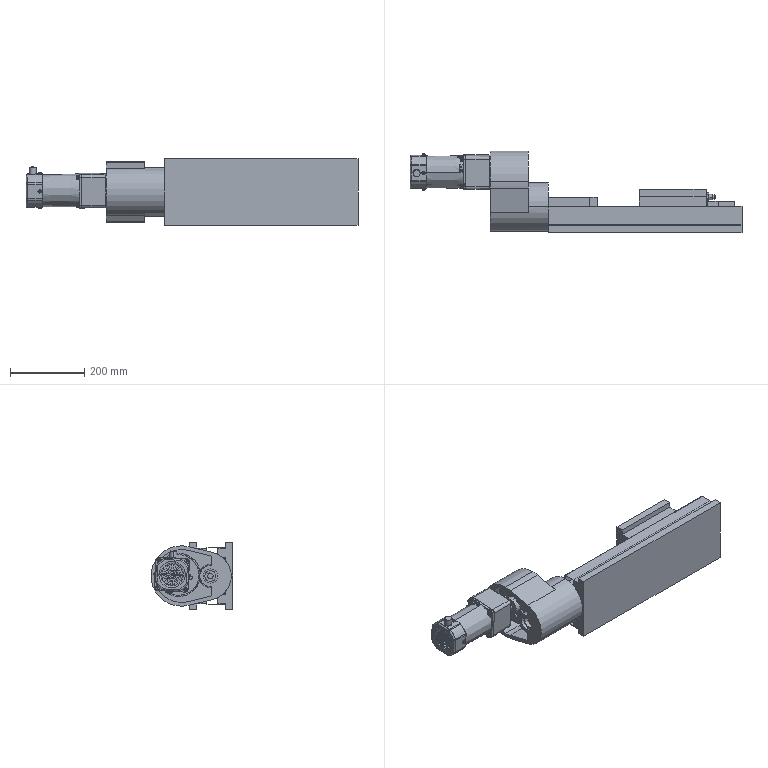Assembly | SolidWorks | mm | 44 component files | 275 solids | 3085 faces | box 892.1 x 219.71 x 180 mm | volume 7665810 mm3 | cylinder 1026 | sphere 846 | plane 710 | spline 244 | cone 147 | torus 112 | commonest cylinder face diameters 115.5 x76 108.75 x75 2 x53 20 x52 15 x47 39 x38 50.25 x36 57 x36
Bill of materials:
BallScrew | 1 |  | Long, slender cylindrical shaft. Both ends step down to smaller diameters, and there is a band of evenly spaced circumferential grooves partway along its length.
BearingHousing | 1 |  | Appears to be two separate prismatic bodies. One is a thin rectangular block with a round through-hole and a recessed or open lower region. The other is a solid rectangular box next to it.
ConnectingFlange | 2 |  | Long, straight, thin-walled profile with a Z/S-shaped cross-section. Two parallel flanges are joined by a web, with rounded bends at the corners.
ConnectingSeat | 1 |  | Rectangular block with a large cylindrical through-bore. Seen from the end, it has a stepped T-like profile: a wider flange section on one side and a narrower body around the bore.
CopperGasket | 1 |  | Thin flat rectangular plate with four small round through-holes in a rectangular pattern, set in from the edges.
CountersunkScrewM5X20 | 6 |  | Stepped cylindrical pin. A larger-diameter head transitions to a smaller shank with a chamfered end, and there is a polygonal socket recess in the head end face.
CountersunkScrewM8x4 | 4 |  | Stepped cylindrical pin with a short, larger-diameter head and a longer, smaller-diameter shank that has a chamfered tip.
CouplingSleeve | 1 |  | Cylindrical tube or sleeve with a coaxial bore. There is a small rectangular notch or keyway-like cut in the bore wall along its length.
DeepGrooveBallBearing16002 | 5 |  | Ring-shaped assembly-like body with an outer ring, a wide inner ring with a central bore, and a single circular row of balls between them.
DeepGrooveBallBearing6204 | 1 |  | Thin-section ring body with narrow outer and inner rings, a single circular row of balls between them, and a large central opening.
EndCap | 1 |  | Bracket-like body: a flat rectangular plate with four corner holes and a rectangular slot, with a hollow rectangular frame extending from one face. Curved surfaces are visible inside the frame.
Gearbox | 1 |  | Stepped solid with a teardrop/obround (cam-like) profile: a large rounded lobe joined to a smaller rounded end by tangent flats. It has a small through-hole near the smaller end and a thickness step between regions.
GearboxLargeGear | 1 |  | Straight-toothed spur gear with many teeth, a central round bore, six round holes evenly spaced around the bore, and a cylindrical hub sticking out from one face.
GearboxSmallGear | 1 |  | Small spur gear (pinion) with roughly thirty-some straight teeth, a plain central round bore, and a cylindrical hub on one side about half as long as the toothed section.
GearShaft | 1 |  | Long, slender, plain cylindrical rod with a small rectangular slot or flat cut near each end.
HexSocketScrewM6X15 | 1 |  | Fastener-like solid shaped like a socket head cap screw: a cylindrical head with a hexagonal socket and a plain cylindrical shank with a chamfered tip.
NutSeat | 1 |  | Solid rectangular block with one round hole in one of its smaller end faces.
OilCup | 1 |  | Turned part with a hexagonal flange section: a short cylindrical collar on one end, a hex section, a cylindrical body, a smaller stepped section with a chamfer, and a small pointed conical tip.
OriginalWasher | 2 |  | Thin-walled cylindrical ring or band with a rectangular cross-section.
ParallelKey5x5x25 | 1 |  | Prism with a stadium-shaped (obround) outline: an elongated block with two flat parallel faces and fully rounded ends.
RoundNut | 2 |  | Thick flat annular washer or spacer ring with a rectangular cross-section.
RoundNutLockWasher15 | 2 |  | Thin annular disc with a conical (dished) profile, like a cone-shaped spring washer.
SealingAnvil | 1 |  | Flat plate of constant thickness made of a tall rectangular strip joined to a shorter, wider rectangular section that has one round through-hole.
SealingFelt | 1 |  | Annular washer or ring with a central bore and the outer edge chamfered on both faces, giving a tapered edge profile in side view.
ShaftRetainingRing | 1 |  | Flat annular ring (plain washer-like disc): thin circular disc with a concentric circular through-hole and flat parallel faces.
StepperMotor | 1 |  | Elongated unit that looks like a motor with a gearbox: a cylindrical main body with a rounded end cap at one end and a square-flanged housing at the other, ending in a protruding output shaft with a keyway and key, on a circular pilot boss. A short cylindrical stub sticks out sideways near the end-cap end.
WorkPlatform | 1 |  | Rectangular plate with two parallel rectangular ribs running its full length on one face, set in from the edges. The plate has six small through-holes in two columns of three; the middle hole of each column looks slightly larger.
X-AxisSupportBase | 1 |  | Long, thin bar of constant cross-section. One face of the flat strip has two outer rectangular lips and a slightly lower central land between them, separated from each lip by a narrow slot with a small rounded root.
Mates:
1. coincident | X-AxisSupportBase-1 face at (-277, 20, 115) dir (-1, 0, 0) | ConnectingFlange-3 face at (-277, 70, 48.661) dir (-1, 0, 0)
2. coincident | X-AxisSupportBase-1 face at (503, 0, 49.398) dir (0, 0, -1) | ConnectingFlange-3 face at (0, 20, 49.398) dir (0, 0, 1)
3. parallel | X-AxisSupportBase-1 face at (0, 0, 0) dir (0, -1, 0) | WorkPlatform-1 face at (56.772, 116.74, 0) dir (0, 1, 0)
4. parallel | X-AxisSupportBase-1 face at (-277, 20, 115) dir (0, 0, 1) | WorkPlatform-1 face at (171.772, 116.74, 115) dir (0, 0, 1)
5. coincident | X-AxisSupportBase-1 face at (0, 20, 0) dir (0, 1, 0) | ConnectingSeat-1 face at (-166, 20, 46.072) dir (0, -1, 0)
6. coincident | X-AxisSupportBase-1 face at (-277, 20, 115) dir (-1, 0, 0) | ConnectingSeat-1 face at (-277, 40, 0) dir (-1, 0, 0)
7. coincident | ConnectingSeat-1 face at (-277, 40, 0) dir (-1, 0, 0) | Gearbox-1 face at (-277, 69.2, 0) dir (1, 0, 0)
8. concentric | Gearbox-1 face at (-302, 60.219, 0) dir (1, 0, 0) r 25.57 | GearboxSmallGear-1 face at (-323.574, 60.219, 0) dir (-1, 0, 0) r 7.5
9. coincident | Gearbox-1 plane at (-277, 0, 0) dir (0, 0, -1) | assembly plane at (0, 0, 0) dir (0, 0, 1)
10. concentric | BallScrew-1 face at (263, 60.219, 0) dir (1, 0, 0) r 7.5 | BearingHousing-1 face at (194.019, 60.219, 0) dir (-1, 0, 0) r 10.5
11. concentric | BallScrew-1 face at (263, 60.219, 0) dir (-1, 0, 0) r 10 | NutSeat-1 face at (-31.284, 60.219, 0) dir (1, 0, 0) r 10
12. coincident | BallScrew-1 sketch segment at (103, 60.219, 0) dir (1, 0, 0) r 10 | NutSeat-1 sketch segment at (103, 60.219, 0) dir (1, 0, 0) r 10
13. concentric | ConnectingSeat-1 face at (-281, 60.219, 0) dir (1, 0, 0) r 25.57 | DeepGrooveBallBearing16002-1 face at (-186, 60.219, 0) dir (-1, 0, 0) r 23.5
14. coincident | ConnectingSeat-1 face at (-166, 40, 0) dir (1, 0, 0) | DeepGrooveBallBearing16002-2 face at (-166, 82.472, 6.559) dir (1, 0, 0)
15. concentric | BallScrew-1 face at (-250, 60.219, 0) dir (1, 0, 0) r 6.215 | CouplingSleeve-1 face at (-286.5, 60.219, 0) dir (1, 0, 0) r 8.58
16. distance | GearShaft-1 face at (-277, 60.219, 0) dir (1, 0, 0) | BallScrew-1 face at (-272, 60.219, 0) dir (-1, 0, 0)
17. coincident | GearboxSmallGear-1 face at (-413, 60.219, 0) dir (-1, 0, 0) | GearShaft-1 face at (-413, 60.219, 0) dir (-1, 0, 0)
18. coincident | GearShaft-1 face at (-282, 56.727, -0.07861) dir (0, 0.7323, 0.681) | ParallelKey5x5x25-1 face at (-14.748, 51.96, 5.047) dir (0, -0.7323, -0.681)
19. coincident | BallScrew-1 face at (-265, 56.727, -0.07861) dir (0, 0.7323, 0.681) | ParallelKey5x5x25-1 face at (-14.748, 51.96, 5.047) dir (0, -0.7323, -0.681)
20. coincident | GearShaft-1 face at (-282, 56.727, -0.07861) dir (0, -0.681, 0.7323) | ParallelKey5x5x25-1 edge at (-280.428, 56.727, -0.07861) dir (1, 0, 0)
21. coincident | BallScrew-1 face at (-265, 56.727, -0.07861) dir (0, -0.681, 0.7323) | ParallelKey5x5x25-1 edge at (-280.428, 56.727, -0.07861) dir (1, 0, 0)
22. tangent | GearShaft-1 face at (-282, 101.228, -44.098) dir (1, 0, 0) | ParallelKey5x5x25-1 face at (-279.134, 58.6, 1.663) dir (0, -0.681, 0.7323) r 2.866
23. concentric | BallScrew-1 face at (-250, 60.219, 0) dir (1, 0, 0) r 6.215 | Gearbox-1 face at (-292, 60.219, 0) dir (1, 0, 0) r 18.564
24. concentric | Gearbox-1 face at (-398.993, 60.219, 0) dir (-1, 0, 0) r 15 | GearShaft-1 edge at (-413, 60.219, 0) dir (-1, 0, 0) r 7.5
25. coincident | BallScrew-1 edge at (-249.5, 60.219, 0) dir (1, 0, 0) r 6.215 | CouplingSleeve-1 face at (-249.5, 60.219, 0) dir (1, 0, 0)
26. concentric | BallScrew-1 face at (263, 60.219, 0) dir (-1, 0, 0) r 10 | RoundNutLockWasher15-1 edge at (-186, 60.219, 0) dir (-1, 0, 0) r 10.006
27. concentric | BallScrew-1 face at (263, 60.219, 0) dir (-1, 0, 0) r 10 | RoundNut-1 face at (-196.75, 60.219, 0) dir (1, 0, 0) r 19.5
28. coincident | RoundNut-1 edge at (-187.75, 60.219, 0) dir (-1, 0, 0) r 19.5 | RoundNutLockWasher15-1 edge at (-187.75, 60.219, 0) dir (-1, 0, 0) r 19.5
29. coincident | DeepGrooveBallBearing16002-1 face at (-186, 52.87, -16.212) dir (-1, 0, 0) | RoundNutLockWasher15-1 face at (-186, 80.498, 0) dir (1, 0, 0)
30. coincident | DeepGrooveBallBearing16002-1 face at (-179, 52.168, -17.76) dir (1, 0, 0) | OriginalWasher-1 face at (-179, 59.486, -0.1318) dir (-1, 0, 0)
31. coincident | DeepGrooveBallBearing16002-2 face at (-173, 77.293, 5.033) dir (-1, 0, 0) | OriginalWasher-1 face at (-173, 59.486, -0.1318) dir (1, 0, 0)
32. concentric | BallScrew-1 face at (263, 60.219, 0) dir (-1, 0, 0) r 10 | OriginalWasher-1 face at (-176, 60.219, 0) dir (1, 0, 0) r 16.311
33. coincident | Gearbox-1 face at (-331, 60.219, 0) dir (-1, 0, 0) | DeepGrooveBallBearing16002-4 face at (-331, 83.419, 0) dir (-1, 0, 0)
34. concentric | BallScrew-1 face at (263, 60.219, 0) dir (-1, 0, 0) r 10 | SealingAnvil-1 face at (-146, 60.219, 0) dir (-1, 0, 0) r 10
35. parallel | X-AxisSupportBase-1 face at (0, 20, 0) dir (0, 1, 0) | SealingAnvil-1 face at (-146, 39.822, -46.072) dir (0, 1, 0)
36. coincident | X-AxisSupportBase-1 face at (0, 20, 0) dir (0, 1, 0) | SealingAnvil-1 edge at (-166, 20, 46.072) dir (0, 0, -1)
37. coincident | ConnectingSeat-1 face at (-166, 40, 0) dir (1, 0, 0) | SealingAnvil-1 face at (-166, 0, 0) dir (-1, 0, 0)
38. concentric | BallScrew-1 face at (263, 60.219, 0) dir (-1, 0, 0) r 10 | DeepGrooveBallBearing16002-5 face at (203.498, 60.219, 0) dir (-1, 0, 0) r 11.01
39. concentric | BallScrew-1 face at (263, 60.219, 0) dir (1, 0, 0) r 7.5 | DeepGrooveBallBearing16002-6 face at (216.498, 60.219, 0) dir (-1, 0, 0) r 11.01
40. concentric | BallScrew-1 face at (263, 60.219, 0) dir (1, 0, 0) r 7.5 | OriginalWasher-2 face at (156.152, 60.219, 0) dir (1, 0, 0) r 19.557
41. coincident | DeepGrooveBallBearing16002-5 face at (153.152, 66.274, 18.536) dir (1, 0, 0) | OriginalWasher-2 face at (153.152, 59.486, -0.1289) dir (-1, 0, 0)
42. coincident | DeepGrooveBallBearing16002-6 face at (159.152, 75.449, 9.213) dir (-1, 0, 0) | OriginalWasher-2 face at (159.152, 59.486, -0.1289) dir (1, 0, 0)
43. coincident | DeepGrooveBallBearing16002-6 face at (166.152, 76.904, 10.093) dir (1, 0, 0) | RoundNutLockWasher15-2 face at (166.152, 63.673, 19.982) dir (-1, 0, 0)
44. concentric | RoundNutLockWasher15-2 edge at (167.752, 60.219, 0) dir (1, 0, 0) r 10.006 | RoundNut-2 face at (167.902, 60.219, 0) dir (1, 0, 0) r 10
45. coincident | RoundNutLockWasher15-2 face at (167.902, 60.219, 0) dir (-1, 0, 0) r 1554.999 | RoundNut-2 edge at (167.902, 60.219, 0) dir (-1, 0, 0) r 19.5
46. concentric | Gearbox-1 face at (-425, 60.219, 0) dir (-1, 0, 0) r 19.092 | DeepGrooveBallBearing6204-2 face at (-413, 60.219, 0) dir (-1, 0, 0) r 15
47. coincident | Gearbox-1 face at (-406, 60.219, 0) dir (1, 0, 0) | DeepGrooveBallBearing6204-2 face at (-406, 80.67, -3.201) dir (1, 0, 0)
48. parallel | GearboxSmallGear-1 face at (-396, 57.853, 1.33) dir (0, 0.8717, -0.4901) | GearShaft-1 face at (-388.806, 48.864, -14.657) dir (0, 0.8717, -0.4901)
49. coincident | GearboxSmallGear-1 face at (-366, 60.219, 0) dir (1, 0, 0) | ShaftRetainingRing-1 edge at (-366, 60.219, 0) dir (1, 0, 0) r 15.026
50. coincident | GearboxSmallGear-1 face at (-413, 60.219, 0) dir (-1, 0, 0) | DeepGrooveBallBearing6204-2 edge at (-413, 60.219, 0) dir (-1, 0, 0) r 15.3
51. parallel | GearboxSmallGear-1 face at (-413, 60.219, 0) dir (-1, 0, 0) | GearboxLargeGear-4 face at (-410, 145.203, 2.782) dir (-1, 0, 0)
52. concentric | StepperMotor-2 face at (-426.5, 145.203, 2.782) dir (1, 0, 0) r 7.5 | GearboxLargeGear-4 face at (-318, 145.203, 2.782) dir (-1, 0, 0) r 14.069
53. coincident | Gearbox-1 face at (-434, 138.635, 0) dir (-1, 0, 0) | StepperMotor-2 face at (-434, 163.177, 3.733) dir (1, 0, 0)
54. coincident | GearboxLargeGear-4 face at (-376, 122.44, 26.591) dir (1, 0, 0) | CountersunkScrewM5X20-1 edge at (-376, 122.44, 26.591) dir (1, 0, 0) r 7.5
55. concentric | GearboxLargeGear-4 face at (-376, 122.44, 26.591) dir (1, 0, 0) r 7.5 | CountersunkScrewM5X20-1 face at (-362, 122.44, 26.591) dir (-1, 0, 0) r 7.5
56. coincident | WorkPlatform-1 face at (56.772, 96.74, 0) dir (0, -1, 0) | CopperGasket-1 face at (-3, 96.74, 0) dir (0, 1, 0)
57. concentric | WorkPlatform-1 face at (86.571, 106.74, -20.473) dir (0, 1, 0) r 4.017 | CountersunkScrewM8x4-2 face at (86.571, 87.74, -20.473) dir (0, 1, 0) r 2.25
58. concentric | WorkPlatform-1 face at (86.571, 58.74, 20.473) dir (0, 1, 0) r 2.271 | CountersunkScrewM8x4-4 face at (86.571, 87.74, 20.473) dir (0, 1, 0) r 2.25
59. concentric | WorkPlatform-1 face at (26.973, 58.74, 20.473) dir (0, 1, 0) r 2.271 | CountersunkScrewM8x4-3 face at (26.973, 87.74, 20.473) dir (0, 1, 0) r 2.25
60. coincident | GearboxSmallGear-1 face at (-396, 60.219, 0) dir (-1, 0, 0) | GearboxLargeGear-4 face at (-396, 145.203, 2.782) dir (-1, 0, 0)
61. gear | GearboxSmallGear-1 sketch segment at (-396, 60.219, 0) dir (-1, 0, 0) r 26.846 | GearboxLargeGear-4 sketch segment at (-396, 145.203, 2.782) dir (-1, 0, 0) r 56.581
62. coincident | BearingHousing-1 edge at (178.784, 84.114, -27.5) dir (0, 0, 1) | EndCap-2 face at (178.784, 77.114, 0) dir (1, 0, 0)
63. coincident | BearingHousing-1 face at (-54.961, 84.114, 27.5) dir (0, 1, 0) | EndCap-2 face at (158.784, 84.114, -27.5) dir (0, 1, 0)
64. coincident | BearingHousing-1 face at (-54.961, 85.587, 27.5) dir (0, 0, 1) | EndCap-2 face at (158.784, 84.114, 27.5) dir (0, 0, 1)
65. concentric | X-AxisSupportBase-1 face at (157.679, 36, 37.292) dir (0, -1, 0) r 2.542 | EndCap-2 face at (157.679, 32.078, 37.292) dir (0, 1, 0) r 2.542
66. concentric | BallScrew-1 face at (263, 60.219, 0) dir (-1, 0, 0) r 10 | RoundNut-2 face at (167.902, 60.219, 0) dir (1, 0, 0) r 19.5
67. concentric | WorkPlatform-1 face at (141.772, 96.052, -63.122) dir (1, 0, 0) r 8.316 | OilCup-1 face at (154.272, 96.052, -63.122) dir (-1, 0, 0) r 8.316
68. coincident | WorkPlatform-1 face at (146.772, 44.74, 0) dir (1, 0, 0) | OilCup-1 edge at (146.772, 90.18, -72.283) dir (0, 0.9989, -0.04636)
69. concentric | GearShaft-1 face at (-277, 60.219, 0) dir (-1, 0, 0) r 7.5 | ShaftRetainingRing-1 face at (-363, 60.219, 0) dir (-1, 0, 0) r 7.5